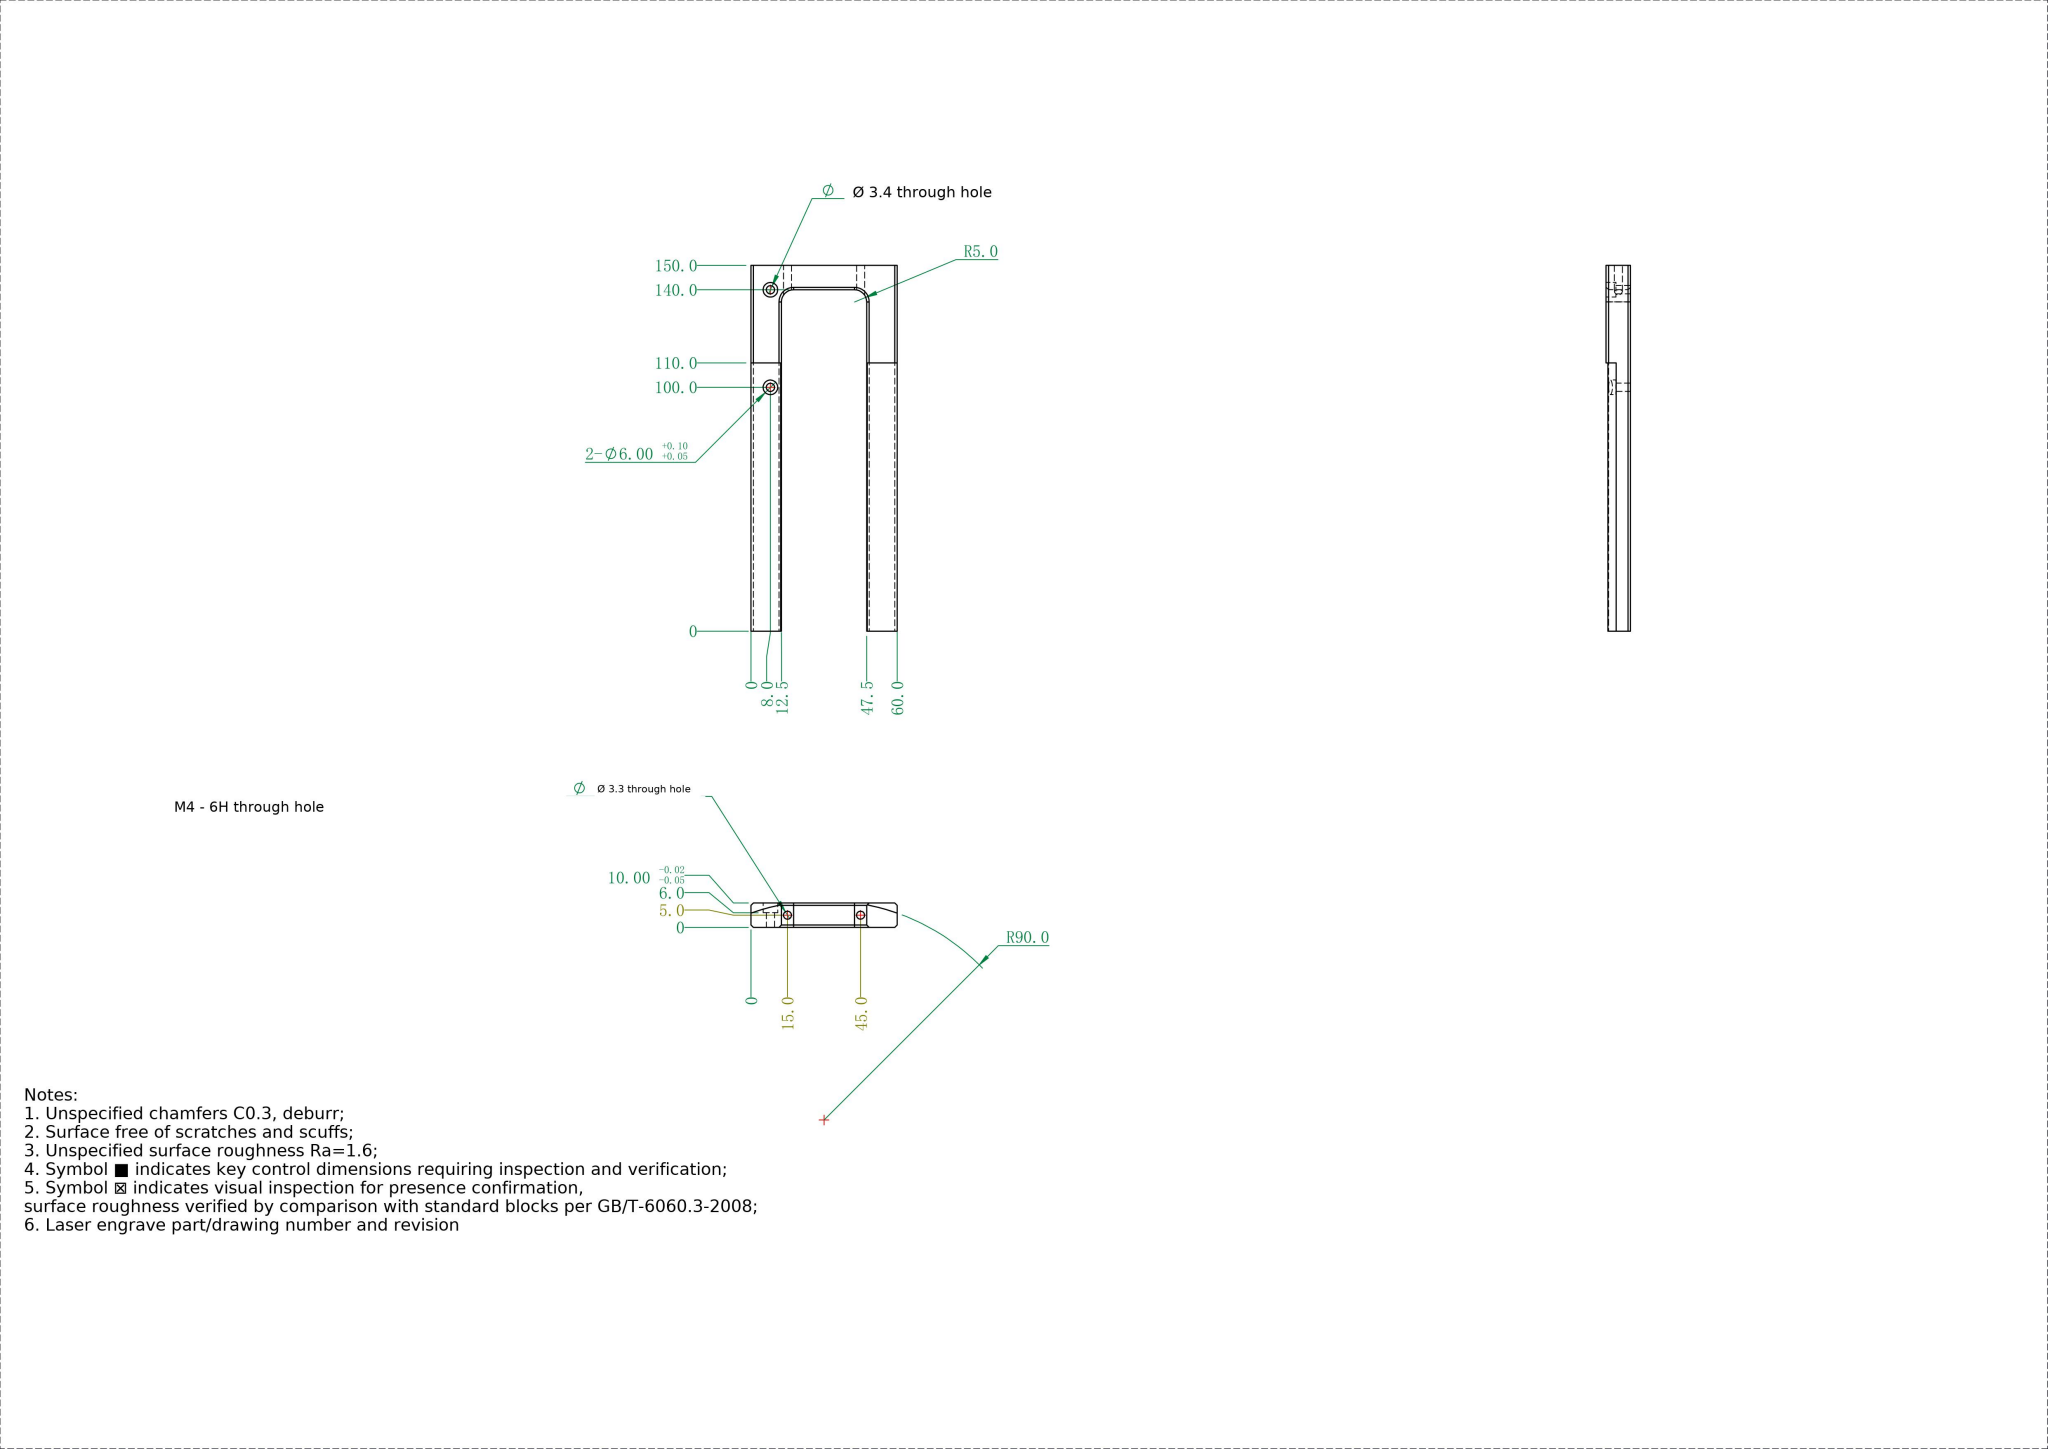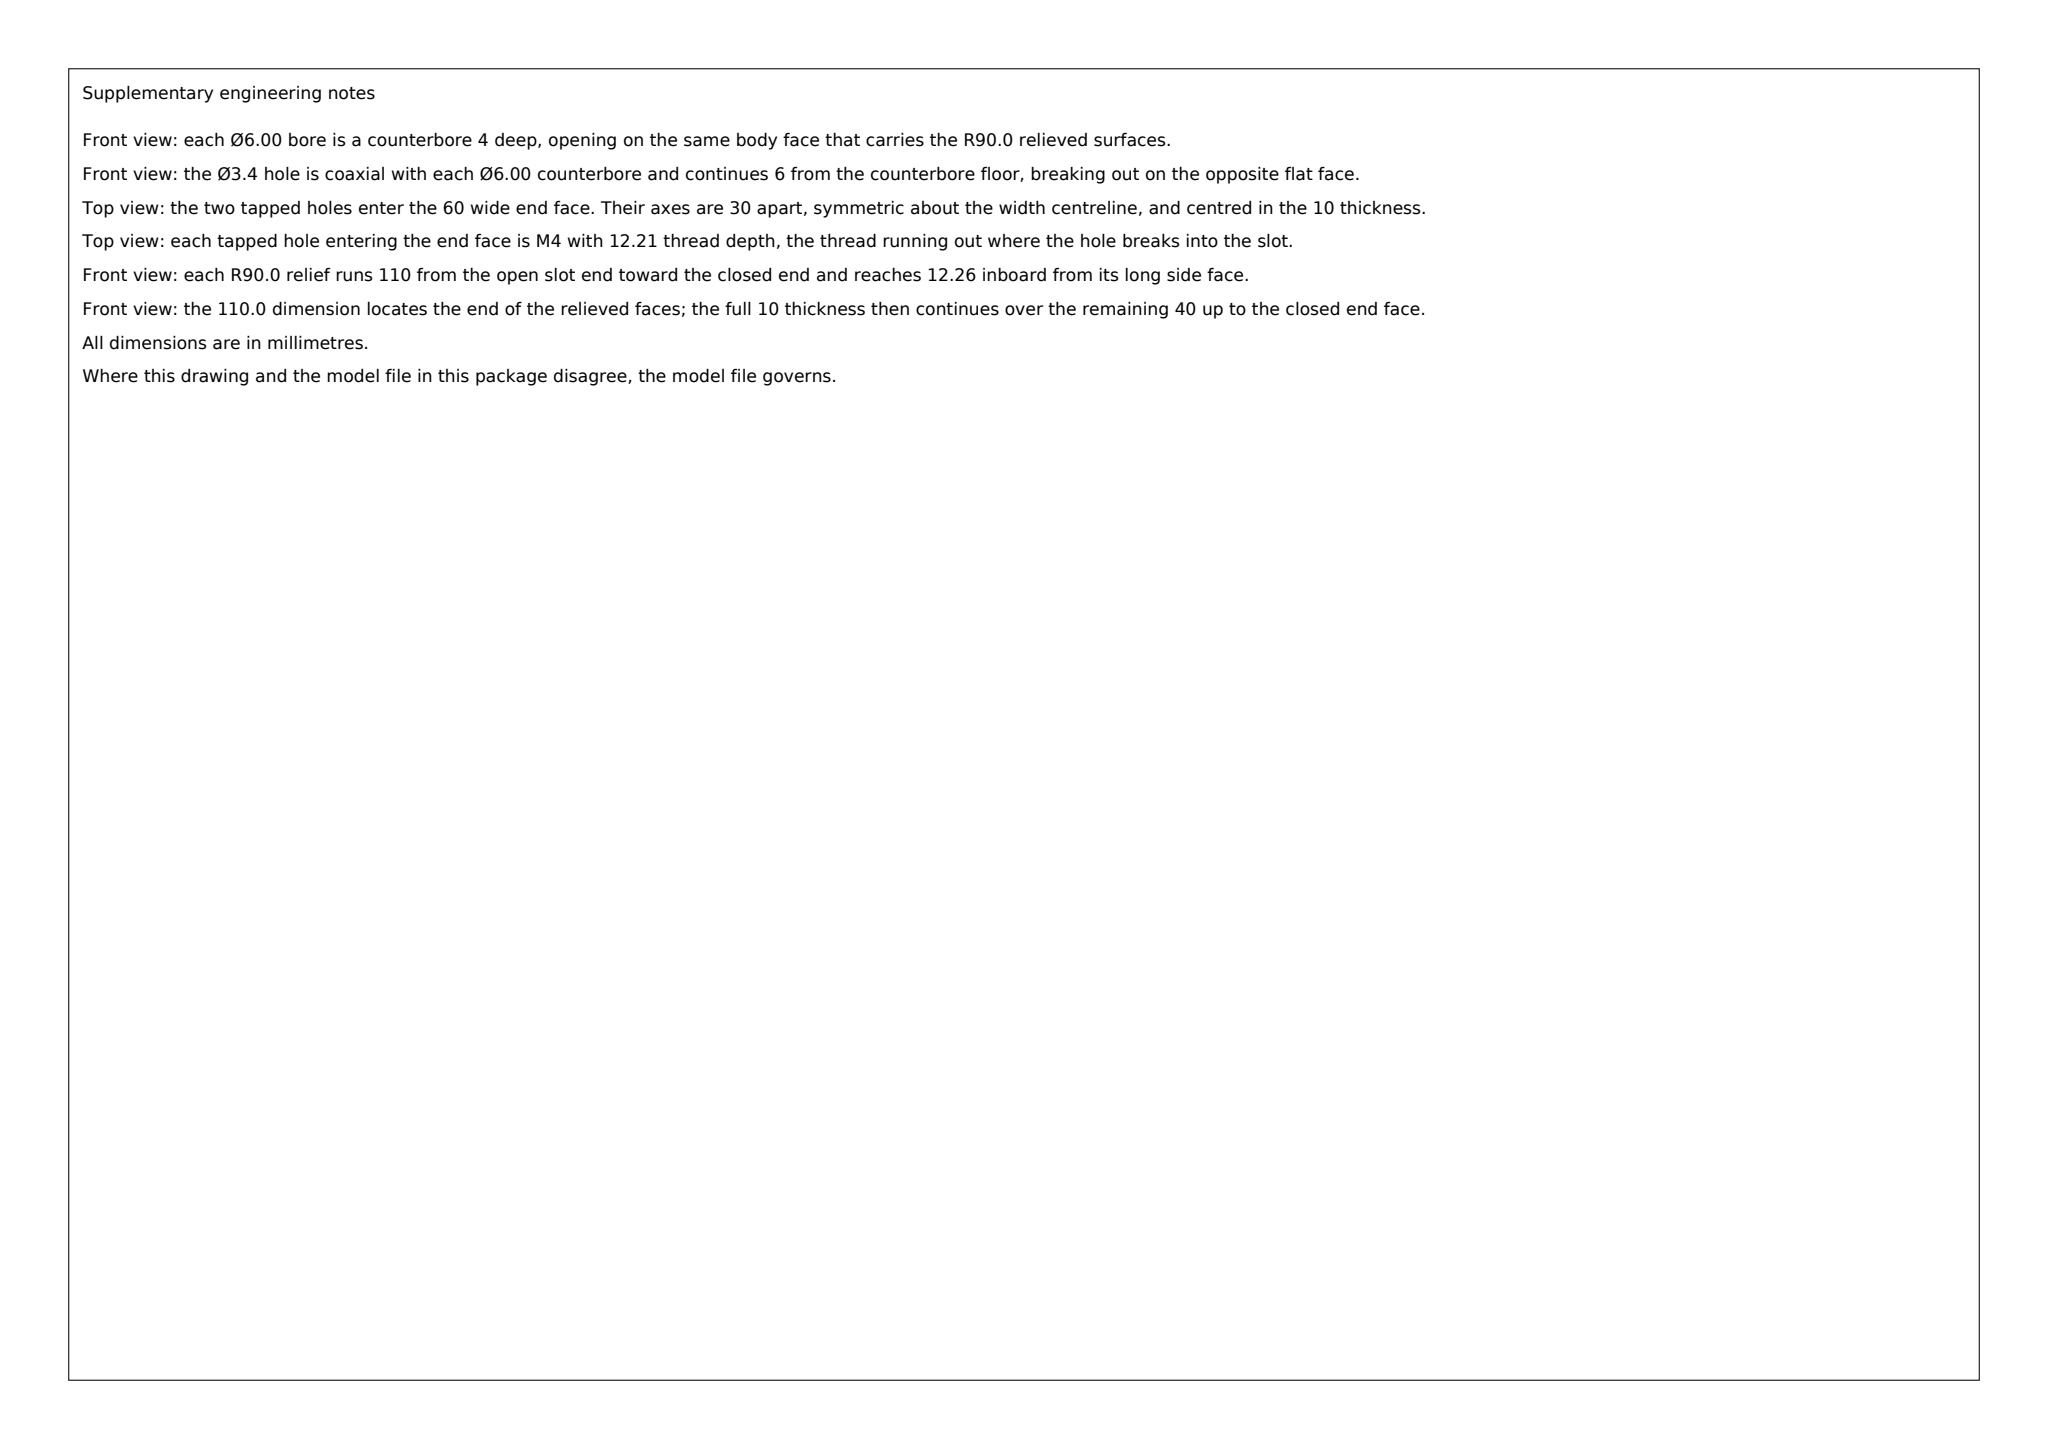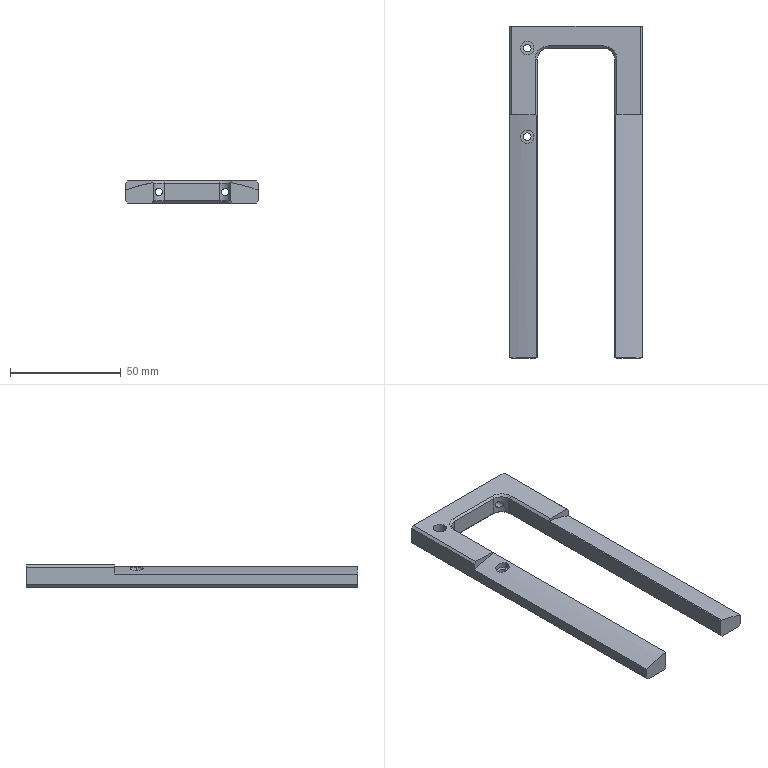Part | SolidWorks | mm | 1 solid | 44 faces | box 60 x 150 x 10 mm | volume 33993 mm3 | plane 24 | cylinder 16 | cone 4 | commonest cylinder face diameters 3.3 x4 3.4 x4 6 x4 180 x2 10 x2